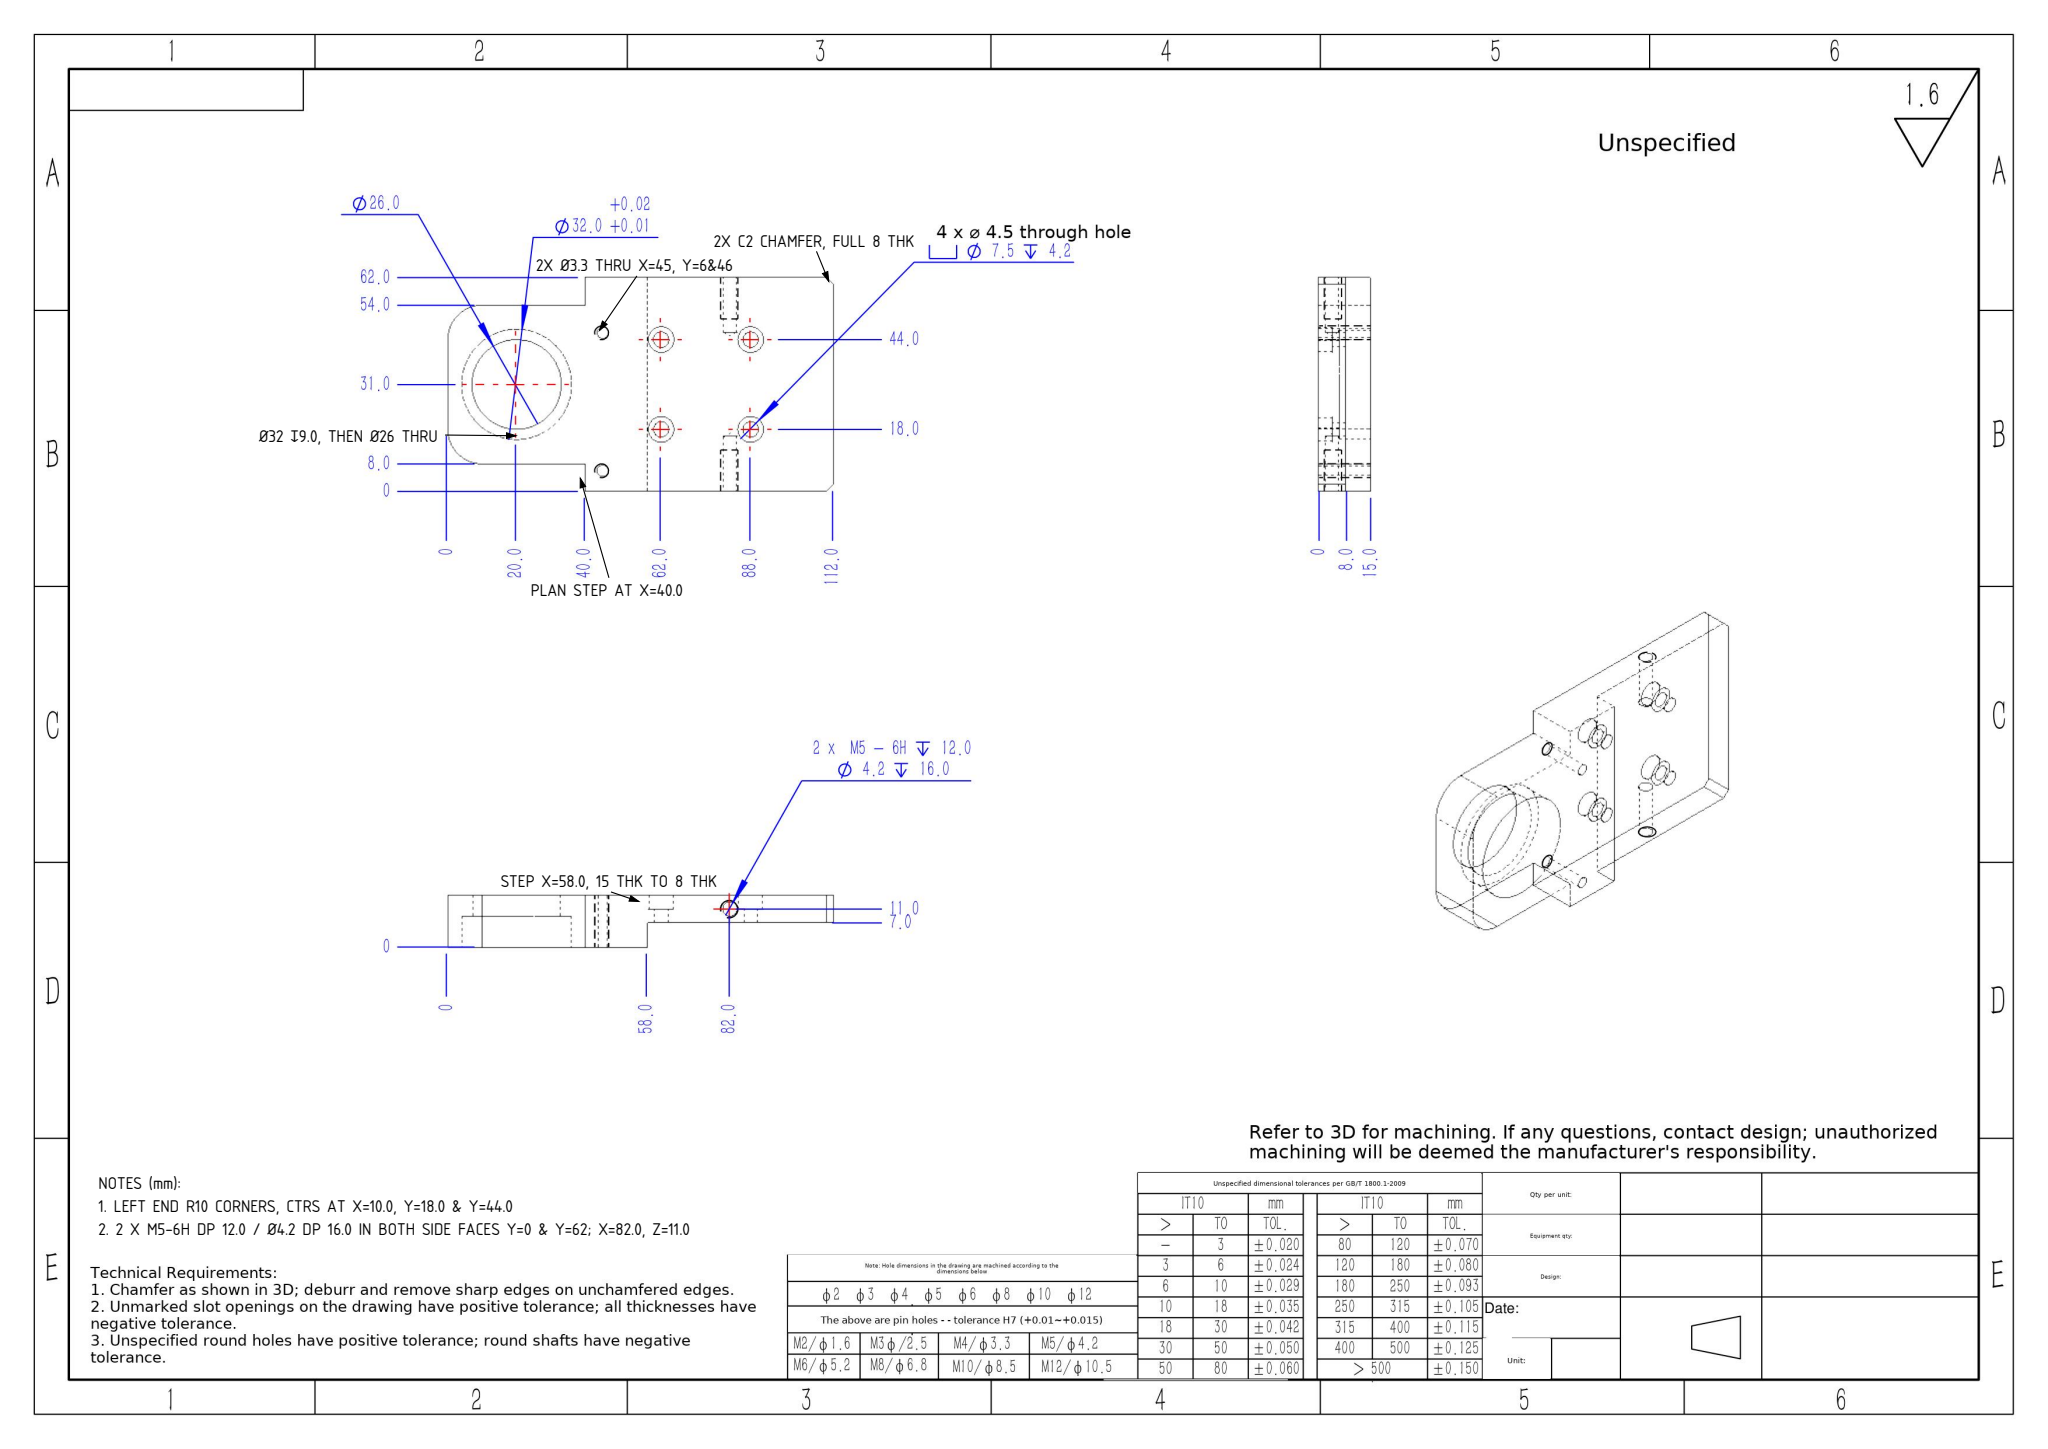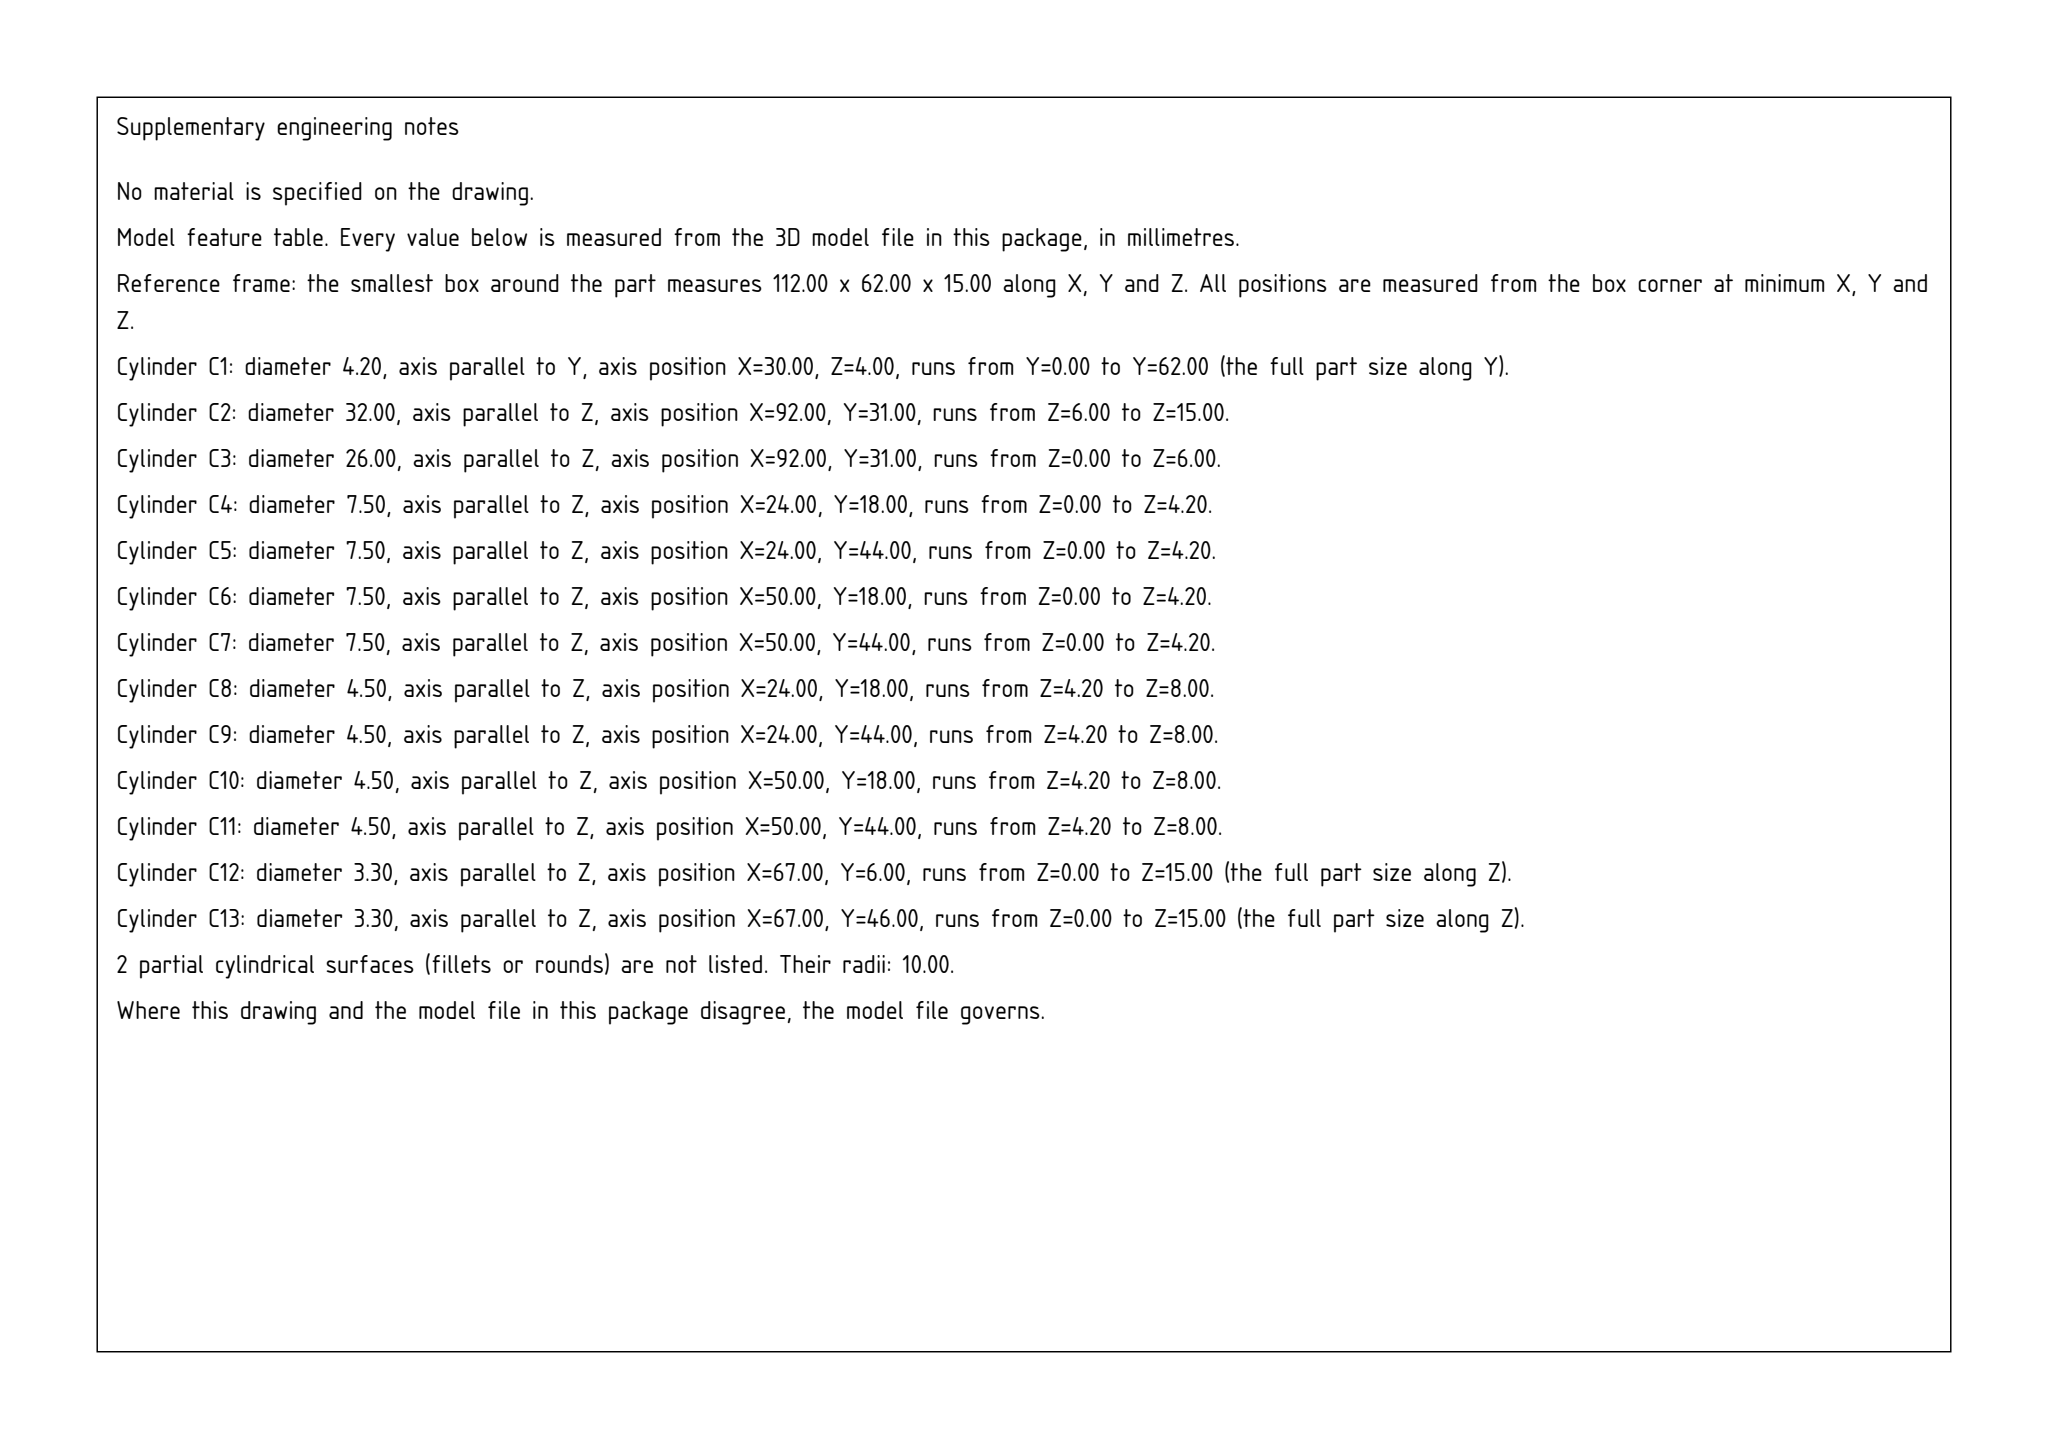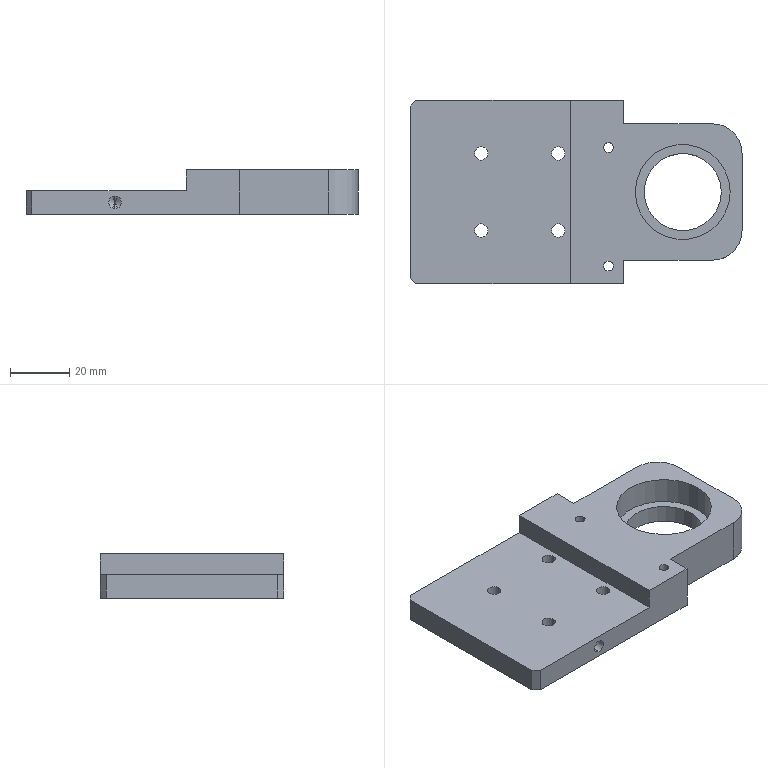Part | SolidWorks | mm | 1 solid | 53 faces | box 112 x 62 x 15 mm | volume 58329 mm3 | cylinder 30 | plane 19 | cone 4 | commonest cylinder face diameters 7.5 x8 4.5 x8 3.3 x4 4.2 x4 32 x2 26 x2 20 x2
Drawing notes:
PLAN STEP AT X=40.0: Y=8.0-54.0 LEFT OF STEP, Y=0-62.0 RIGHT | from the solid: x-planes 72.0 x2 (=112-72=40); y-planes 0, 8.0, 54.0, 62.0
THK STEP AT X=58.0: 15.0 THK AT X<58.0, 8.0 THK AT X>58.0 | from the solid: x-plane 54.0 (=112-54=58); z-planes 0/8.0/15.0; Ø4.5 hole 3.8 + Ø7.5 CBORE 4.2 = 8.0 thk
LEFT END R10 CORNERS, CTRS AT X=10.0, Y=18.0 & Y=44.0 | from the solid: Ø20 z-axis cyls at (102,18) & (102,44) len 15 = full thk; 112-102=10
Ø32.0 DP 9.0 FROM NEAR FACE, THEN Ø26.0 THRU; CL X=20.0, Y=31.0 | from the solid: cyl dia 32 axis Z at (92,31) len 9.0 + dia 26 len 6.0 = 15 thru; 112-92=20
2 X Ø3.3 THRU AT X=45.0, Y=6.0 & Y=46.0 | from the solid: cyl dia 3.3 axis Z at (67,6) & (67,46) len 15 = thru; 112-67=45
2 X M5-6H DP 12.0 / Ø4.2 DP 16.0 IN BOTH SIDE FACES Y=0 & Y=62; X=82.0, Z=11.0 | from the solid: cyl dia 4.2 axis Y at x=30 (=112-30=82), z=4.0 (=15-4=11), len 16 from y=0 and y=62; cone 118 deg
2 X 45° CHAMFER 2.0 X 2.0, FULL 8.0 THICKNESS (Z=0 TO 8.0), AT THIN-END CORNERS X=112.0/Y=0 AND X=112.0/Y=62.0 | from the solid: inclined_planes: angle_to_xyz_axes [45.0,45.0,90.0], bbox_from [0,0,0] and [0,60,0], size [2.0,2.0,8.0] (two 45° faces spanning 2 mm in X and Y over the 8 mm thin section)